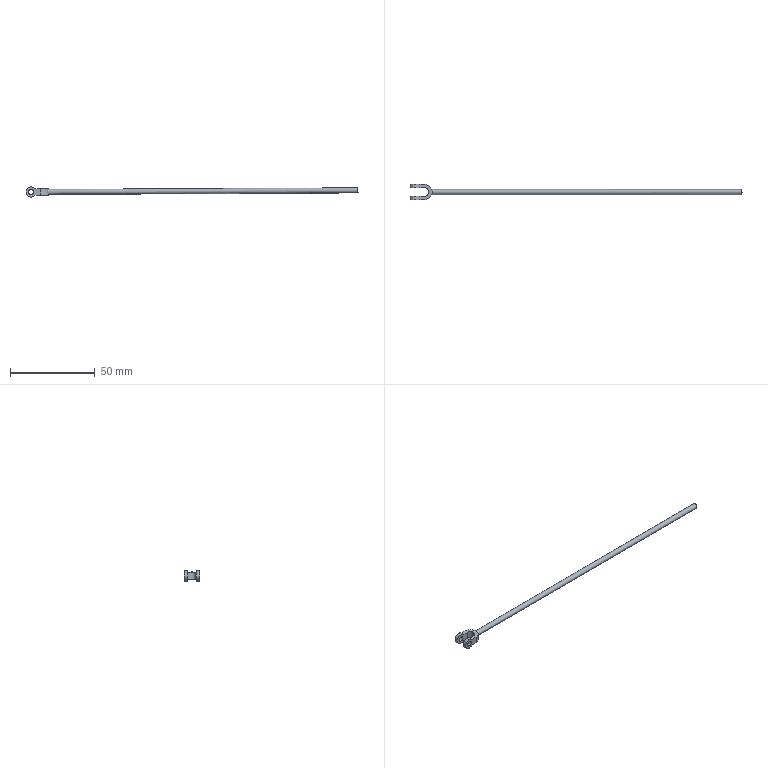Component | NX | LINK_5 | 1 solid | 14 faces | volume 1507 mm3 | cylinder 7 | plane 7 | commonest cylinder face diameters 3 x3 6 x2 9 x1 5 x1